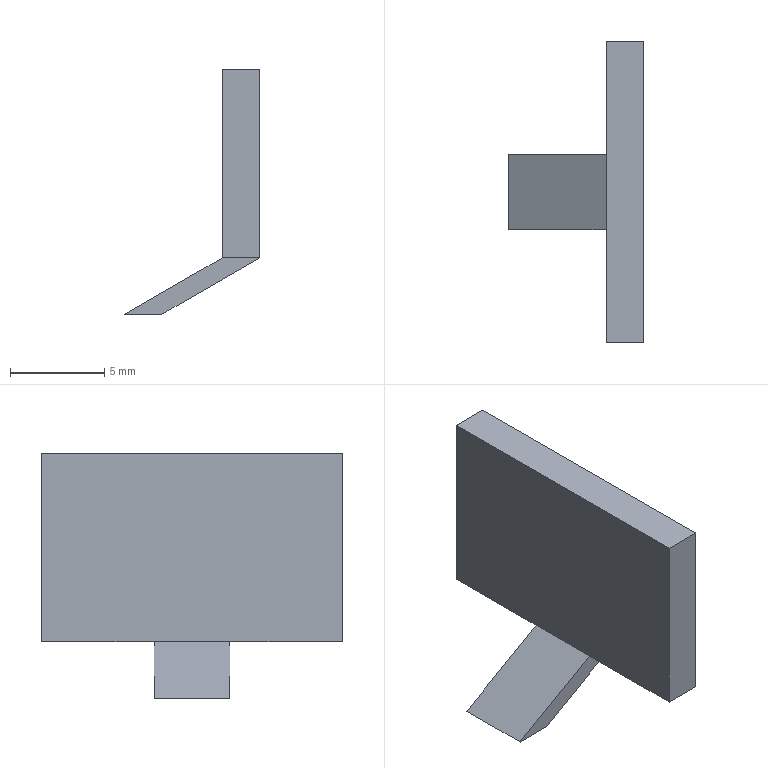Component | NX | GRIPPER_21 | 1 solid | 12 faces | box 7.2 x 16 x 12.99 mm | volume 344 mm3 | plane 12
STEP:
#1=CARTESIAN_POINT('',(0.,0.,0.));
#2=DIRECTION('',(0.,0.,1.));
#3=DIRECTION('',(1.,0.,0.));
#4=AXIS2_PLACEMENT_3D('',#1,#2,#3);
#5=CARTESIAN_POINT('',(26.071,12.637,119.668));
#6=VERTEX_POINT('',#5);
#7=CARTESIAN_POINT('',(24.071,12.637,119.668));
#8=VERTEX_POINT('',#7);
#9=CARTESIAN_POINT('',(26.071,12.637,119.668));
#10=DIRECTION('',(-1.,0.,0.));
#11=VECTOR('',#10,1.);
#12=LINE('',#9,#11);
#13=CARTESIAN_POINT('',(24.071,6.637,119.668));
#14=DIRECTION('',(0.,0.,1.));
#15=DIRECTION('',(-1.,0.,0.));
#16=AXIS2_PLACEMENT_3D('',#13,#14,#15);
#17=PLANE('',#16);
#18=CARTESIAN_POINT('',(-2.,-6.));
#19=DIRECTION('',(1.,0.));
#20=VECTOR('',#19,1.);
#21=LINE('',#18,#20);
#22=(GEOMETRIC_REPRESENTATION_CONTEXT(2)PARAMETRIC_REPRESENTATION_CONTEXT()REPRESENTATION_CONTEXT('',''));
#23=DEFINITIONAL_REPRESENTATION('',(#21),#22);
#24=PCURVE('',#17,#23);
#25=CARTESIAN_POINT('',(26.071,12.637,119.668));
#26=DIRECTION('',(0.,-1.,0.));
#27=DIRECTION('',(1.,0.,0.));
#28=AXIS2_PLACEMENT_3D('',#25,#26,#27);
#29=PLANE('',#28);
#30=CARTESIAN_POINT('',(0.,0.));
#31=DIRECTION('',(-1.,0.));
#32=VECTOR('',#31,1.);
#33=LINE('',#30,#32);
#34=(GEOMETRIC_REPRESENTATION_CONTEXT(2)PARAMETRIC_REPRESENTATION_CONTEXT()REPRESENTATION_CONTEXT('',''));
#35=DEFINITIONAL_REPRESENTATION('',(#33),#34);
#36=PCURVE('',#29,#35);
#37=SURFACE_CURVE('',#12,(#24,#36),.PCURVE_S1.);
#38=EDGE_CURVE('',#6,#8,#37,.T.);
#39=ORIENTED_EDGE('',*,*,#38,.F.);
#40=CARTESIAN_POINT('',(26.071,6.637,119.668));
#41=VERTEX_POINT('',#40);
#42=CARTESIAN_POINT('',(26.071,6.637,119.668));
#43=DIRECTION('',(0.,1.,0.));
#44=VECTOR('',#43,1.);
#45=LINE('',#42,#44);
#46=CARTESIAN_POINT('',(-2.,0.));
#47=DIRECTION('',(0.,-1.));
#48=VECTOR('',#47,1.);
#49=LINE('',#46,#48);
#50=(GEOMETRIC_REPRESENTATION_CONTEXT(2)PARAMETRIC_REPRESENTATION_CONTEXT()REPRESENTATION_CONTEXT('',''));
#51=DEFINITIONAL_REPRESENTATION('',(#49),#50);
#52=PCURVE('',#17,#51);
#53=CARTESIAN_POINT('',(26.071,6.637,119.668));
#54=DIRECTION('',(-1.,0.,0.));
#55=DIRECTION('',(0.,-1.,0.));
#56=AXIS2_PLACEMENT_3D('',#53,#54,#55);
#57=PLANE('',#56);
#58=CARTESIAN_POINT('',(0.,0.));
#59=DIRECTION('',(-1.,0.));
#60=VECTOR('',#59,1.);
#61=LINE('',#58,#60);
#62=(GEOMETRIC_REPRESENTATION_CONTEXT(2)PARAMETRIC_REPRESENTATION_CONTEXT()REPRESENTATION_CONTEXT('',''));
#63=DEFINITIONAL_REPRESENTATION('',(#61),#62);
#64=PCURVE('',#57,#63);
#65=SURFACE_CURVE('',#45,(#52,#64),.PCURVE_S1.);
#66=EDGE_CURVE('',#41,#6,#65,.T.);
#67=ORIENTED_EDGE('',*,*,#66,.F.);
#68=CARTESIAN_POINT('',(24.071,6.637,119.668));
#69=VERTEX_POINT('',#68);
#70=CARTESIAN_POINT('',(24.071,6.637,119.668));
#71=DIRECTION('',(1.,0.,-0.));
#72=VECTOR('',#71,1.);
#73=LINE('',#70,#72);
#74=CARTESIAN_POINT('',(0.,0.));
#75=DIRECTION('',(-1.,0.));
#76=VECTOR('',#75,1.);
#77=LINE('',#74,#76);
#78=(GEOMETRIC_REPRESENTATION_CONTEXT(2)PARAMETRIC_REPRESENTATION_CONTEXT()REPRESENTATION_CONTEXT('',''));
#79=DEFINITIONAL_REPRESENTATION('',(#77),#78);
#80=PCURVE('',#17,#79);
#81=CARTESIAN_POINT('',(26.071,6.637,119.668));
#82=DIRECTION('',(0.,-1.,0.));
#83=DIRECTION('',(1.,0.,0.));
#84=AXIS2_PLACEMENT_3D('',#81,#82,#83);
#85=PLANE('',#84);
#86=CARTESIAN_POINT('',(-2.,0.));
#87=DIRECTION('',(1.,-0.));
#88=VECTOR('',#87,1.);
#89=LINE('',#86,#88);
#90=(GEOMETRIC_REPRESENTATION_CONTEXT(2)PARAMETRIC_REPRESENTATION_CONTEXT()REPRESENTATION_CONTEXT('',''));
#91=DEFINITIONAL_REPRESENTATION('',(#89),#90);
#92=PCURVE('',#85,#91);
#93=SURFACE_CURVE('',#73,(#80,#92),.PCURVE_S1.);
#94=EDGE_CURVE('',#69,#41,#93,.T.);
#95=ORIENTED_EDGE('',*,*,#94,.F.);
#96=CARTESIAN_POINT('',(24.071,6.637,119.668));
#97=DIRECTION('',(0.,1.,0.));
#98=VECTOR('',#97,1.);
#99=LINE('',#96,#98);
#100=CARTESIAN_POINT('',(0.,0.));
#101=DIRECTION('',(0.,-1.));
#102=VECTOR('',#101,1.);
#103=LINE('',#100,#102);
#104=(GEOMETRIC_REPRESENTATION_CONTEXT(2)PARAMETRIC_REPRESENTATION_CONTEXT()REPRESENTATION_CONTEXT('',''));
#105=DEFINITIONAL_REPRESENTATION('',(#103),#104);
#106=PCURVE('',#17,#105);
#107=CARTESIAN_POINT('',(24.071,6.637,129.668));
#108=DIRECTION('',(1.,0.,0.));
#109=DIRECTION('',(-0.,0.,1.));
#110=AXIS2_PLACEMENT_3D('',#107,#108,#109);
#111=PLANE('',#110);
#112=CARTESIAN_POINT('',(-10.,0.));
#113=DIRECTION('',(0.,-1.));
#114=VECTOR('',#113,1.);
#115=LINE('',#112,#114);
#116=(GEOMETRIC_REPRESENTATION_CONTEXT(2)PARAMETRIC_REPRESENTATION_CONTEXT()REPRESENTATION_CONTEXT('',''));
#117=DEFINITIONAL_REPRESENTATION('',(#115),#116);
#118=PCURVE('',#111,#117);
#119=SURFACE_CURVE('',#99,(#106,#118),.PCURVE_S1.);
#120=EDGE_CURVE('',#69,#8,#119,.T.);
#121=ORIENTED_EDGE('',*,*,#120,.T.);
#122=EDGE_LOOP('',(#39,#67,#95,#121));
#123=FACE_BOUND('',#122,.T.);
#124=ADVANCED_FACE('',(#123),#17,.F.);
#125=CARTESIAN_POINT('',(26.071,22.637,119.668));
#126=VERTEX_POINT('',#125);
#127=CARTESIAN_POINT('',(26.071,22.637,129.668));
#128=VERTEX_POINT('',#127);
#129=CARTESIAN_POINT('',(26.071,22.637,119.668));
#130=DIRECTION('',(0.,0.,1.));
#131=VECTOR('',#130,1.);
#132=LINE('',#129,#131);
#133=CARTESIAN_POINT('',(-16.,0.));
#134=DIRECTION('',(0.,1.));
#135=VECTOR('',#134,1.);
#136=LINE('',#133,#135);
#137=(GEOMETRIC_REPRESENTATION_CONTEXT(2)PARAMETRIC_REPRESENTATION_CONTEXT()REPRESENTATION_CONTEXT('',''));
#138=DEFINITIONAL_REPRESENTATION('',(#136),#137);
#139=PCURVE('',#57,#138);
#140=CARTESIAN_POINT('',(26.071,22.637,119.668));
#141=DIRECTION('',(0.,-1.,0.));
#142=DIRECTION('',(1.,0.,0.));
#143=AXIS2_PLACEMENT_3D('',#140,#141,#142);
#144=PLANE('',#143);
#145=CARTESIAN_POINT('',(0.,0.));
#146=DIRECTION('',(0.,1.));
#147=VECTOR('',#146,1.);
#148=LINE('',#145,#147);
#149=(GEOMETRIC_REPRESENTATION_CONTEXT(2)PARAMETRIC_REPRESENTATION_CONTEXT()REPRESENTATION_CONTEXT('',''));
#150=DEFINITIONAL_REPRESENTATION('',(#148),#149);
#151=PCURVE('',#144,#150);
#152=SURFACE_CURVE('',#132,(#139,#151),.PCURVE_S1.);
#153=EDGE_CURVE('',#126,#128,#152,.T.);
#154=ORIENTED_EDGE('',*,*,#153,.T.);
#155=CARTESIAN_POINT('',(26.071,6.637,129.668));
#156=VERTEX_POINT('',#155);
#157=CARTESIAN_POINT('',(26.071,6.637,129.668));
#158=DIRECTION('',(0.,1.,0.));
#159=VECTOR('',#158,1.);
#160=LINE('',#157,#159);
#161=CARTESIAN_POINT('',(0.,10.));
#162=DIRECTION('',(-1.,0.));
#163=VECTOR('',#162,1.);
#164=LINE('',#161,#163);
#165=(GEOMETRIC_REPRESENTATION_CONTEXT(2)PARAMETRIC_REPRESENTATION_CONTEXT()REPRESENTATION_CONTEXT('',''));
#166=DEFINITIONAL_REPRESENTATION('',(#164),#165);
#167=PCURVE('',#57,#166);
#168=CARTESIAN_POINT('',(26.071,6.637,129.668));
#169=DIRECTION('',(-0.,0.,-1.));
#170=DIRECTION('',(1.,0.,-0.));
#171=AXIS2_PLACEMENT_3D('',#168,#169,#170);
#172=PLANE('',#171);
#173=CARTESIAN_POINT('',(0.,0.));
#174=DIRECTION('',(0.,-1.));
#175=VECTOR('',#174,1.);
#176=LINE('',#173,#175);
#177=(GEOMETRIC_REPRESENTATION_CONTEXT(2)PARAMETRIC_REPRESENTATION_CONTEXT()REPRESENTATION_CONTEXT('',''));
#178=DEFINITIONAL_REPRESENTATION('',(#176),#177);
#179=PCURVE('',#172,#178);
#180=SURFACE_CURVE('',#160,(#167,#179),.PCURVE_S1.);
#181=EDGE_CURVE('',#156,#128,#180,.T.);
#182=ORIENTED_EDGE('',*,*,#181,.F.);
#183=CARTESIAN_POINT('',(26.071,6.637,119.668));
#184=DIRECTION('',(0.,0.,1.));
#185=VECTOR('',#184,1.);
#186=LINE('',#183,#185);
#187=CARTESIAN_POINT('',(0.,0.));
#188=DIRECTION('',(0.,1.));
#189=VECTOR('',#188,1.);
#190=LINE('',#187,#189);
#191=(GEOMETRIC_REPRESENTATION_CONTEXT(2)PARAMETRIC_REPRESENTATION_CONTEXT()REPRESENTATION_CONTEXT('',''));
#192=DEFINITIONAL_REPRESENTATION('',(#190),#191);
#193=PCURVE('',#57,#192);
#194=CARTESIAN_POINT('',(0.,0.));
#195=DIRECTION('',(0.,1.));
#196=VECTOR('',#195,1.);
#197=LINE('',#194,#196);
#198=(GEOMETRIC_REPRESENTATION_CONTEXT(2)PARAMETRIC_REPRESENTATION_CONTEXT()REPRESENTATION_CONTEXT('',''));
#199=DEFINITIONAL_REPRESENTATION('',(#197),#198);
#200=PCURVE('',#85,#199);
#201=SURFACE_CURVE('',#186,(#193,#200),.PCURVE_S1.);
#202=EDGE_CURVE('',#41,#156,#201,.T.);
#203=ORIENTED_EDGE('',*,*,#202,.F.);
#204=ORIENTED_EDGE('',*,*,#66,.T.);
#205=CARTESIAN_POINT('',(26.071,16.637,119.668));
#206=VERTEX_POINT('',#205);
#207=CARTESIAN_POINT('',(26.071,12.637,119.668));
#208=DIRECTION('',(0.,1.,0.));
#209=VECTOR('',#208,1.);
#210=LINE('',#207,#209);
#211=CARTESIAN_POINT('',(-6.,0.));
#212=DIRECTION('',(-1.,0.));
#213=VECTOR('',#212,1.);
#214=LINE('',#211,#213);
#215=(GEOMETRIC_REPRESENTATION_CONTEXT(2)PARAMETRIC_REPRESENTATION_CONTEXT()REPRESENTATION_CONTEXT('',''));
#216=DEFINITIONAL_REPRESENTATION('',(#214),#215);
#217=PCURVE('',#57,#216);
#218=CARTESIAN_POINT('',(20.871,12.637,116.674));
#219=DIRECTION('',(-0.4989,0.,0.8667));
#220=DIRECTION('',(-0.8667,0.,-0.4989));
#221=AXIS2_PLACEMENT_3D('',#218,#219,#220);
#222=PLANE('',#221);
#223=CARTESIAN_POINT('',(-6.,0.));
#224=DIRECTION('',(0.,-1.));
#225=VECTOR('',#224,1.);
#226=LINE('',#223,#225);
#227=(GEOMETRIC_REPRESENTATION_CONTEXT(2)PARAMETRIC_REPRESENTATION_CONTEXT()REPRESENTATION_CONTEXT('',''));
#228=DEFINITIONAL_REPRESENTATION('',(#226),#227);
#229=PCURVE('',#222,#228);
#230=SURFACE_CURVE('',#210,(#217,#229),.PCURVE_S1.);
#231=EDGE_CURVE('',#6,#206,#230,.T.);
#232=ORIENTED_EDGE('',*,*,#231,.T.);
#233=CARTESIAN_POINT('',(26.071,6.637,119.668));
#234=DIRECTION('',(0.,1.,0.));
#235=VECTOR('',#234,1.);
#236=LINE('',#233,#235);
#237=CARTESIAN_POINT('',(0.,0.));
#238=DIRECTION('',(-1.,0.));
#239=VECTOR('',#238,1.);
#240=LINE('',#237,#239);
#241=(GEOMETRIC_REPRESENTATION_CONTEXT(2)PARAMETRIC_REPRESENTATION_CONTEXT()REPRESENTATION_CONTEXT('',''));
#242=DEFINITIONAL_REPRESENTATION('',(#240),#241);
#243=PCURVE('',#57,#242);
#244=CARTESIAN_POINT('',(24.071,6.637,119.668));
#245=DIRECTION('',(0.,0.,1.));
#246=DIRECTION('',(-1.,0.,0.));
#247=AXIS2_PLACEMENT_3D('',#244,#245,#246);
#248=PLANE('',#247);
#249=CARTESIAN_POINT('',(-2.,0.));
#250=DIRECTION('',(0.,-1.));
#251=VECTOR('',#250,1.);
#252=LINE('',#249,#251);
#253=(GEOMETRIC_REPRESENTATION_CONTEXT(2)PARAMETRIC_REPRESENTATION_CONTEXT()REPRESENTATION_CONTEXT('',''));
#254=DEFINITIONAL_REPRESENTATION('',(#252),#253);
#255=PCURVE('',#248,#254);
#256=SURFACE_CURVE('',#236,(#243,#255),.PCURVE_S1.);
#257=EDGE_CURVE('',#206,#126,#256,.T.);
#258=ORIENTED_EDGE('',*,*,#257,.T.);
#259=EDGE_LOOP('',(#154,#182,#203,#204,#232,#258));
#260=FACE_BOUND('',#259,.T.);
#261=ADVANCED_FACE('',(#260),#57,.F.);
#262=CARTESIAN_POINT('',(24.071,22.637,129.668));
#263=VERTEX_POINT('',#262);
#264=CARTESIAN_POINT('',(26.071,22.637,129.668));
#265=DIRECTION('',(-1.,0.,0.));
#266=VECTOR('',#265,1.);
#267=LINE('',#264,#266);
#268=CARTESIAN_POINT('',(0.,-16.));
#269=DIRECTION('',(-1.,0.));
#270=VECTOR('',#269,1.);
#271=LINE('',#268,#270);
#272=(GEOMETRIC_REPRESENTATION_CONTEXT(2)PARAMETRIC_REPRESENTATION_CONTEXT()REPRESENTATION_CONTEXT('',''));
#273=DEFINITIONAL_REPRESENTATION('',(#271),#272);
#274=PCURVE('',#172,#273);
#275=CARTESIAN_POINT('',(0.,10.));
#276=DIRECTION('',(-1.,0.));
#277=VECTOR('',#276,1.);
#278=LINE('',#275,#277);
#279=(GEOMETRIC_REPRESENTATION_CONTEXT(2)PARAMETRIC_REPRESENTATION_CONTEXT()REPRESENTATION_CONTEXT('',''));
#280=DEFINITIONAL_REPRESENTATION('',(#278),#279);
#281=PCURVE('',#144,#280);
#282=SURFACE_CURVE('',#267,(#274,#281),.PCURVE_S1.);
#283=EDGE_CURVE('',#128,#263,#282,.T.);
#284=ORIENTED_EDGE('',*,*,#283,.T.);
#285=CARTESIAN_POINT('',(24.071,6.637,129.668));
#286=VERTEX_POINT('',#285);
#287=CARTESIAN_POINT('',(24.071,6.637,129.668));
#288=DIRECTION('',(0.,1.,0.));
#289=VECTOR('',#288,1.);
#290=LINE('',#287,#289);
#291=CARTESIAN_POINT('',(-2.,0.));
#292=DIRECTION('',(0.,-1.));
#293=VECTOR('',#292,1.);
#294=LINE('',#291,#293);
#295=(GEOMETRIC_REPRESENTATION_CONTEXT(2)PARAMETRIC_REPRESENTATION_CONTEXT()REPRESENTATION_CONTEXT('',''));
#296=DEFINITIONAL_REPRESENTATION('',(#294),#295);
#297=PCURVE('',#172,#296);
#298=CARTESIAN_POINT('',(0.,0.));
#299=DIRECTION('',(0.,-1.));
#300=VECTOR('',#299,1.);
#301=LINE('',#298,#300);
#302=(GEOMETRIC_REPRESENTATION_CONTEXT(2)PARAMETRIC_REPRESENTATION_CONTEXT()REPRESENTATION_CONTEXT('',''));
#303=DEFINITIONAL_REPRESENTATION('',(#301),#302);
#304=PCURVE('',#111,#303);
#305=SURFACE_CURVE('',#290,(#297,#304),.PCURVE_S1.);
#306=EDGE_CURVE('',#286,#263,#305,.T.);
#307=ORIENTED_EDGE('',*,*,#306,.F.);
#308=CARTESIAN_POINT('',(26.071,6.637,129.668));
#309=DIRECTION('',(-1.,0.,0.));
#310=VECTOR('',#309,1.);
#311=LINE('',#308,#310);
#312=CARTESIAN_POINT('',(0.,0.));
#313=DIRECTION('',(-1.,0.));
#314=VECTOR('',#313,1.);
#315=LINE('',#312,#314);
#316=(GEOMETRIC_REPRESENTATION_CONTEXT(2)PARAMETRIC_REPRESENTATION_CONTEXT()REPRESENTATION_CONTEXT('',''));
#317=DEFINITIONAL_REPRESENTATION('',(#315),#316);
#318=PCURVE('',#172,#317);
#319=CARTESIAN_POINT('',(0.,10.));
#320=DIRECTION('',(-1.,0.));
#321=VECTOR('',#320,1.);
#322=LINE('',#319,#321);
#323=(GEOMETRIC_REPRESENTATION_CONTEXT(2)PARAMETRIC_REPRESENTATION_CONTEXT()REPRESENTATION_CONTEXT('',''));
#324=DEFINITIONAL_REPRESENTATION('',(#322),#323);
#325=PCURVE('',#85,#324);
#326=SURFACE_CURVE('',#311,(#318,#325),.PCURVE_S1.);
#327=EDGE_CURVE('',#156,#286,#326,.T.);
#328=ORIENTED_EDGE('',*,*,#327,.F.);
#329=ORIENTED_EDGE('',*,*,#181,.T.);
#330=EDGE_LOOP('',(#284,#307,#328,#329));
#331=FACE_BOUND('',#330,.T.);
#332=ADVANCED_FACE('',(#331),#172,.F.);
#333=CARTESIAN_POINT('',(24.071,22.637,119.668));
#334=VERTEX_POINT('',#333);
#335=CARTESIAN_POINT('',(24.071,22.637,129.668));
#336=DIRECTION('',(0.,0.,-1.));
#337=VECTOR('',#336,1.);
#338=LINE('',#335,#337);
#339=CARTESIAN_POINT('',(0.,-16.));
#340=DIRECTION('',(-1.,0.));
#341=VECTOR('',#340,1.);
#342=LINE('',#339,#341);
#343=(GEOMETRIC_REPRESENTATION_CONTEXT(2)PARAMETRIC_REPRESENTATION_CONTEXT()REPRESENTATION_CONTEXT('',''));
#344=DEFINITIONAL_REPRESENTATION('',(#342),#343);
#345=PCURVE('',#111,#344);
#346=CARTESIAN_POINT('',(-2.,10.));
#347=DIRECTION('',(0.,-1.));
#348=VECTOR('',#347,1.);
#349=LINE('',#346,#348);
#350=(GEOMETRIC_REPRESENTATION_CONTEXT(2)PARAMETRIC_REPRESENTATION_CONTEXT()REPRESENTATION_CONTEXT('',''));
#351=DEFINITIONAL_REPRESENTATION('',(#349),#350);
#352=PCURVE('',#144,#351);
#353=SURFACE_CURVE('',#338,(#345,#352),.PCURVE_S1.);
#354=EDGE_CURVE('',#263,#334,#353,.T.);
#355=ORIENTED_EDGE('',*,*,#354,.T.);
#356=CARTESIAN_POINT('',(24.071,16.637,119.668));
#357=VERTEX_POINT('',#356);
#358=CARTESIAN_POINT('',(24.071,6.637,119.668));
#359=DIRECTION('',(0.,1.,0.));
#360=VECTOR('',#359,1.);
#361=LINE('',#358,#360);
#362=CARTESIAN_POINT('',(-10.,0.));
#363=DIRECTION('',(0.,-1.));
#364=VECTOR('',#363,1.);
#365=LINE('',#362,#364);
#366=(GEOMETRIC_REPRESENTATION_CONTEXT(2)PARAMETRIC_REPRESENTATION_CONTEXT()REPRESENTATION_CONTEXT('',''));
#367=DEFINITIONAL_REPRESENTATION('',(#365),#366);
#368=PCURVE('',#111,#367);
#369=CARTESIAN_POINT('',(0.,0.));
#370=DIRECTION('',(0.,-1.));
#371=VECTOR('',#370,1.);
#372=LINE('',#369,#371);
#373=(GEOMETRIC_REPRESENTATION_CONTEXT(2)PARAMETRIC_REPRESENTATION_CONTEXT()REPRESENTATION_CONTEXT('',''));
#374=DEFINITIONAL_REPRESENTATION('',(#372),#373);
#375=PCURVE('',#248,#374);
#376=SURFACE_CURVE('',#361,(#368,#375),.PCURVE_S1.);
#377=EDGE_CURVE('',#357,#334,#376,.T.);
#378=ORIENTED_EDGE('',*,*,#377,.F.);
#379=CARTESIAN_POINT('',(24.071,12.637,119.668));
#380=DIRECTION('',(0.,1.,0.));
#381=VECTOR('',#380,1.);
#382=LINE('',#379,#381);
#383=CARTESIAN_POINT('',(-10.,-6.));
#384=DIRECTION('',(0.,-1.));
#385=VECTOR('',#384,1.);
#386=LINE('',#383,#385);
#387=(GEOMETRIC_REPRESENTATION_CONTEXT(2)PARAMETRIC_REPRESENTATION_CONTEXT()REPRESENTATION_CONTEXT('',''));
#388=DEFINITIONAL_REPRESENTATION('',(#386),#387);
#389=PCURVE('',#111,#388);
#390=CARTESIAN_POINT('',(24.071,12.637,119.668));
#391=DIRECTION('',(0.4989,0.,-0.8667));
#392=DIRECTION('',(0.8667,0.,0.4989));
#393=AXIS2_PLACEMENT_3D('',#390,#391,#392);
#394=PLANE('',#393);
#395=CARTESIAN_POINT('',(0.,0.));
#396=DIRECTION('',(0.,-1.));
#397=VECTOR('',#396,1.);
#398=LINE('',#395,#397);
#399=(GEOMETRIC_REPRESENTATION_CONTEXT(2)PARAMETRIC_REPRESENTATION_CONTEXT()REPRESENTATION_CONTEXT('',''));
#400=DEFINITIONAL_REPRESENTATION('',(#398),#399);
#401=PCURVE('',#394,#400);
#402=SURFACE_CURVE('',#382,(#389,#401),.PCURVE_S1.);
#403=EDGE_CURVE('',#8,#357,#402,.T.);
#404=ORIENTED_EDGE('',*,*,#403,.F.);
#405=ORIENTED_EDGE('',*,*,#120,.F.);
#406=CARTESIAN_POINT('',(24.071,6.637,129.668));
#407=DIRECTION('',(0.,0.,-1.));
#408=VECTOR('',#407,1.);
#409=LINE('',#406,#408);
#410=CARTESIAN_POINT('',(0.,0.));
#411=DIRECTION('',(-1.,0.));
#412=VECTOR('',#411,1.);
#413=LINE('',#410,#412);
#414=(GEOMETRIC_REPRESENTATION_CONTEXT(2)PARAMETRIC_REPRESENTATION_CONTEXT()REPRESENTATION_CONTEXT('',''));
#415=DEFINITIONAL_REPRESENTATION('',(#413),#414);
#416=PCURVE('',#111,#415);
#417=CARTESIAN_POINT('',(-2.,10.));
#418=DIRECTION('',(0.,-1.));
#419=VECTOR('',#418,1.);
#420=LINE('',#417,#419);
#421=(GEOMETRIC_REPRESENTATION_CONTEXT(2)PARAMETRIC_REPRESENTATION_CONTEXT()REPRESENTATION_CONTEXT('',''));
#422=DEFINITIONAL_REPRESENTATION('',(#420),#421);
#423=PCURVE('',#85,#422);
#424=SURFACE_CURVE('',#409,(#416,#423),.PCURVE_S1.);
#425=EDGE_CURVE('',#286,#69,#424,.T.);
#426=ORIENTED_EDGE('',*,*,#425,.F.);
#427=ORIENTED_EDGE('',*,*,#306,.T.);
#428=EDGE_LOOP('',(#355,#378,#404,#405,#426,#427));
#429=FACE_BOUND('',#428,.T.);
#430=ADVANCED_FACE('',(#429),#111,.F.);
#431=ORIENTED_EDGE('',*,*,#257,.F.);
#432=CARTESIAN_POINT('',(26.071,16.637,119.668));
#433=DIRECTION('',(-1.,0.,0.));
#434=VECTOR('',#433,1.);
#435=LINE('',#432,#434);
#436=CARTESIAN_POINT('',(-2.,-10.));
#437=DIRECTION('',(1.,0.));
#438=VECTOR('',#437,1.);
#439=LINE('',#436,#438);
#440=(GEOMETRIC_REPRESENTATION_CONTEXT(2)PARAMETRIC_REPRESENTATION_CONTEXT()REPRESENTATION_CONTEXT('',''));
#441=DEFINITIONAL_REPRESENTATION('',(#439),#440);
#442=PCURVE('',#248,#441);
#443=CARTESIAN_POINT('',(26.071,16.637,119.668));
#444=DIRECTION('',(0.,-1.,0.));
#445=DIRECTION('',(1.,0.,0.));
#446=AXIS2_PLACEMENT_3D('',#443,#444,#445);
#447=PLANE('',#446);
#448=CARTESIAN_POINT('',(0.,0.));
#449=DIRECTION('',(-1.,0.));
#450=VECTOR('',#449,1.);
#451=LINE('',#448,#450);
#452=(GEOMETRIC_REPRESENTATION_CONTEXT(2)PARAMETRIC_REPRESENTATION_CONTEXT()REPRESENTATION_CONTEXT('',''));
#453=DEFINITIONAL_REPRESENTATION('',(#451),#452);
#454=PCURVE('',#447,#453);
#455=SURFACE_CURVE('',#435,(#442,#454),.PCURVE_S1.);
#456=EDGE_CURVE('',#206,#357,#455,.T.);
#457=ORIENTED_EDGE('',*,*,#456,.T.);
#458=ORIENTED_EDGE('',*,*,#377,.T.);
#459=CARTESIAN_POINT('',(24.071,22.637,119.668));
#460=DIRECTION('',(1.,0.,-0.));
#461=VECTOR('',#460,1.);
#462=LINE('',#459,#461);
#463=CARTESIAN_POINT('',(0.,-16.));
#464=DIRECTION('',(-1.,0.));
#465=VECTOR('',#464,1.);
#466=LINE('',#463,#465);
#467=(GEOMETRIC_REPRESENTATION_CONTEXT(2)PARAMETRIC_REPRESENTATION_CONTEXT()REPRESENTATION_CONTEXT('',''));
#468=DEFINITIONAL_REPRESENTATION('',(#466),#467);
#469=PCURVE('',#248,#468);
#470=CARTESIAN_POINT('',(-2.,0.));
#471=DIRECTION('',(1.,-0.));
#472=VECTOR('',#471,1.);
#473=LINE('',#470,#472);
#474=(GEOMETRIC_REPRESENTATION_CONTEXT(2)PARAMETRIC_REPRESENTATION_CONTEXT()REPRESENTATION_CONTEXT('',''));
#475=DEFINITIONAL_REPRESENTATION('',(#473),#474);
#476=PCURVE('',#144,#475);
#477=SURFACE_CURVE('',#462,(#469,#476),.PCURVE_S1.);
#478=EDGE_CURVE('',#334,#126,#477,.T.);
#479=ORIENTED_EDGE('',*,*,#478,.T.);
#480=EDGE_LOOP('',(#431,#457,#458,#479));
#481=FACE_BOUND('',#480,.T.);
#482=ADVANCED_FACE('',(#481),#248,.F.);
#483=ORIENTED_EDGE('',*,*,#202,.T.);
#484=ORIENTED_EDGE('',*,*,#327,.T.);
#485=ORIENTED_EDGE('',*,*,#425,.T.);
#486=ORIENTED_EDGE('',*,*,#94,.T.);
#487=EDGE_LOOP('',(#483,#484,#485,#486));
#488=FACE_BOUND('',#487,.T.);
#489=ADVANCED_FACE('',(#488),#85,.T.);
#490=ORIENTED_EDGE('',*,*,#153,.F.);
#491=ORIENTED_EDGE('',*,*,#478,.F.);
#492=ORIENTED_EDGE('',*,*,#354,.F.);
#493=ORIENTED_EDGE('',*,*,#283,.F.);
#494=EDGE_LOOP('',(#490,#491,#492,#493));
#495=FACE_BOUND('',#494,.T.);
#496=ADVANCED_FACE('',(#495),#144,.F.);
#497=CARTESIAN_POINT('',(18.871,16.637,116.674));
#498=VERTEX_POINT('',#497);
#499=CARTESIAN_POINT('',(20.871,16.637,116.674));
#500=VERTEX_POINT('',#499);
#501=CARTESIAN_POINT('',(18.871,16.637,116.674));
#502=DIRECTION('',(1.,0.,0.));
#503=VECTOR('',#502,1.);
#504=LINE('',#501,#503);
#505=CARTESIAN_POINT('',(18.871,12.637,116.674));
#506=DIRECTION('',(0.,0.,1.));
#507=DIRECTION('',(-1.,0.,0.));
#508=AXIS2_PLACEMENT_3D('',#505,#506,#507);
#509=PLANE('',#508);
#510=CARTESIAN_POINT('',(0.,-4.));
#511=DIRECTION('',(-1.,0.));
#512=VECTOR('',#511,1.);
#513=LINE('',#510,#512);
#514=(GEOMETRIC_REPRESENTATION_CONTEXT(2)PARAMETRIC_REPRESENTATION_CONTEXT()REPRESENTATION_CONTEXT('',''));
#515=DEFINITIONAL_REPRESENTATION('',(#513),#514);
#516=PCURVE('',#509,#515);
#517=CARTESIAN_POINT('',(-7.2,-2.993));
#518=DIRECTION('',(1.,0.));
#519=VECTOR('',#518,1.);
#520=LINE('',#517,#519);
#521=(GEOMETRIC_REPRESENTATION_CONTEXT(2)PARAMETRIC_REPRESENTATION_CONTEXT()REPRESENTATION_CONTEXT('',''));
#522=DEFINITIONAL_REPRESENTATION('',(#520),#521);
#523=PCURVE('',#447,#522);
#524=SURFACE_CURVE('',#504,(#516,#523),.PCURVE_S1.);
#525=EDGE_CURVE('',#498,#500,#524,.T.);
#526=ORIENTED_EDGE('',*,*,#525,.T.);
#527=CARTESIAN_POINT('',(20.871,12.637,116.674));
#528=VERTEX_POINT('',#527);
#529=CARTESIAN_POINT('',(20.871,12.637,116.674));
#530=DIRECTION('',(0.,1.,0.));
#531=VECTOR('',#530,1.);
#532=LINE('',#529,#531);
#533=CARTESIAN_POINT('',(-2.,0.));
#534=DIRECTION('',(0.,-1.));
#535=VECTOR('',#534,1.);
#536=LINE('',#533,#535);
#537=(GEOMETRIC_REPRESENTATION_CONTEXT(2)PARAMETRIC_REPRESENTATION_CONTEXT()REPRESENTATION_CONTEXT('',''));
#538=DEFINITIONAL_REPRESENTATION('',(#536),#537);
#539=PCURVE('',#509,#538);
#540=CARTESIAN_POINT('',(0.,0.));
#541=DIRECTION('',(0.,-1.));
#542=VECTOR('',#541,1.);
#543=LINE('',#540,#542);
#544=(GEOMETRIC_REPRESENTATION_CONTEXT(2)PARAMETRIC_REPRESENTATION_CONTEXT()REPRESENTATION_CONTEXT('',''));
#545=DEFINITIONAL_REPRESENTATION('',(#543),#544);
#546=PCURVE('',#222,#545);
#547=SURFACE_CURVE('',#532,(#539,#546),.PCURVE_S1.);
#548=EDGE_CURVE('',#528,#500,#547,.T.);
#549=ORIENTED_EDGE('',*,*,#548,.F.);
#550=CARTESIAN_POINT('',(18.871,12.637,116.674));
#551=VERTEX_POINT('',#550);
#552=CARTESIAN_POINT('',(18.871,12.637,116.674));
#553=DIRECTION('',(1.,0.,0.));
#554=VECTOR('',#553,1.);
#555=LINE('',#552,#554);
#556=CARTESIAN_POINT('',(0.,0.));
#557=DIRECTION('',(-1.,0.));
#558=VECTOR('',#557,1.);
#559=LINE('',#556,#558);
#560=(GEOMETRIC_REPRESENTATION_CONTEXT(2)PARAMETRIC_REPRESENTATION_CONTEXT()REPRESENTATION_CONTEXT('',''));
#561=DEFINITIONAL_REPRESENTATION('',(#559),#560);
#562=PCURVE('',#509,#561);
#563=CARTESIAN_POINT('',(-7.2,-2.993));
#564=DIRECTION('',(1.,0.));
#565=VECTOR('',#564,1.);
#566=LINE('',#563,#565);
#567=(GEOMETRIC_REPRESENTATION_CONTEXT(2)PARAMETRIC_REPRESENTATION_CONTEXT()REPRESENTATION_CONTEXT('',''));
#568=DEFINITIONAL_REPRESENTATION('',(#566),#567);
#569=PCURVE('',#29,#568);
#570=SURFACE_CURVE('',#555,(#562,#569),.PCURVE_S1.);
#571=EDGE_CURVE('',#551,#528,#570,.T.);
#572=ORIENTED_EDGE('',*,*,#571,.F.);
#573=CARTESIAN_POINT('',(18.871,12.637,116.674));
#574=DIRECTION('',(0.,1.,0.));
#575=VECTOR('',#574,1.);
#576=LINE('',#573,#575);
#577=CARTESIAN_POINT('',(0.,0.));
#578=DIRECTION('',(0.,-1.));
#579=VECTOR('',#578,1.);
#580=LINE('',#577,#579);
#581=(GEOMETRIC_REPRESENTATION_CONTEXT(2)PARAMETRIC_REPRESENTATION_CONTEXT()REPRESENTATION_CONTEXT('',''));
#582=DEFINITIONAL_REPRESENTATION('',(#580),#581);
#583=PCURVE('',#509,#582);
#584=CARTESIAN_POINT('',(-6.,0.));
#585=DIRECTION('',(0.,-1.));
#586=VECTOR('',#585,1.);
#587=LINE('',#584,#586);
#588=(GEOMETRIC_REPRESENTATION_CONTEXT(2)PARAMETRIC_REPRESENTATION_CONTEXT()REPRESENTATION_CONTEXT('',''));
#589=DEFINITIONAL_REPRESENTATION('',(#587),#588);
#590=PCURVE('',#394,#589);
#591=SURFACE_CURVE('',#576,(#583,#590),.PCURVE_S1.);
#592=EDGE_CURVE('',#551,#498,#591,.T.);
#593=ORIENTED_EDGE('',*,*,#592,.T.);
#594=EDGE_LOOP('',(#526,#549,#572,#593));
#595=FACE_BOUND('',#594,.T.);
#596=ADVANCED_FACE('',(#595),#509,.F.);
#597=CARTESIAN_POINT('',(20.871,16.637,116.674));
#598=DIRECTION('',(0.8667,0.,0.4989));
#599=VECTOR('',#598,1.);
#600=LINE('',#597,#599);
#601=CARTESIAN_POINT('',(0.,-4.));
#602=DIRECTION('',(-1.,0.));
#603=VECTOR('',#602,1.);
#604=LINE('',#601,#603);
#605=(GEOMETRIC_REPRESENTATION_CONTEXT(2)PARAMETRIC_REPRESENTATION_CONTEXT()REPRESENTATION_CONTEXT('',''));
#606=DEFINITIONAL_REPRESENTATION('',(#604),#605);
#607=PCURVE('',#222,#606);
#608=CARTESIAN_POINT('',(-5.2,-2.993));
#609=DIRECTION('',(0.8667,0.4989));
#610=VECTOR('',#609,1.);
#611=LINE('',#608,#610);
#612=(GEOMETRIC_REPRESENTATION_CONTEXT(2)PARAMETRIC_REPRESENTATION_CONTEXT()REPRESENTATION_CONTEXT('',''));
#613=DEFINITIONAL_REPRESENTATION('',(#611),#612);
#614=PCURVE('',#447,#613);
#615=SURFACE_CURVE('',#600,(#607,#614),.PCURVE_S1.);
#616=EDGE_CURVE('',#500,#206,#615,.T.);
#617=ORIENTED_EDGE('',*,*,#616,.T.);
#618=ORIENTED_EDGE('',*,*,#231,.F.);
#619=CARTESIAN_POINT('',(20.871,12.637,116.674));
#620=DIRECTION('',(0.8667,0.,0.4989));
#621=VECTOR('',#620,1.);
#622=LINE('',#619,#621);
#623=CARTESIAN_POINT('',(0.,0.));
#624=DIRECTION('',(-1.,0.));
#625=VECTOR('',#624,1.);
#626=LINE('',#623,#625);
#627=(GEOMETRIC_REPRESENTATION_CONTEXT(2)PARAMETRIC_REPRESENTATION_CONTEXT()REPRESENTATION_CONTEXT('',''));
#628=DEFINITIONAL_REPRESENTATION('',(#626),#627);
#629=PCURVE('',#222,#628);
#630=CARTESIAN_POINT('',(-5.2,-2.993));
#631=DIRECTION('',(0.8667,0.4989));
#632=VECTOR('',#631,1.);
#633=LINE('',#630,#632);
#634=(GEOMETRIC_REPRESENTATION_CONTEXT(2)PARAMETRIC_REPRESENTATION_CONTEXT()REPRESENTATION_CONTEXT('',''));
#635=DEFINITIONAL_REPRESENTATION('',(#633),#634);
#636=PCURVE('',#29,#635);
#637=SURFACE_CURVE('',#622,(#629,#636),.PCURVE_S1.);
#638=EDGE_CURVE('',#528,#6,#637,.T.);
#639=ORIENTED_EDGE('',*,*,#638,.F.);
#640=ORIENTED_EDGE('',*,*,#548,.T.);
#641=EDGE_LOOP('',(#617,#618,#639,#640));
#642=FACE_BOUND('',#641,.T.);
#643=ADVANCED_FACE('',(#642),#222,.F.);
#644=CARTESIAN_POINT('',(24.071,16.637,119.668));
#645=DIRECTION('',(-0.8667,0.,-0.4989));
#646=VECTOR('',#645,1.);
#647=LINE('',#644,#646);
#648=CARTESIAN_POINT('',(0.,-4.));
#649=DIRECTION('',(-1.,0.));
#650=VECTOR('',#649,1.);
#651=LINE('',#648,#650);
#652=(GEOMETRIC_REPRESENTATION_CONTEXT(2)PARAMETRIC_REPRESENTATION_CONTEXT()REPRESENTATION_CONTEXT('',''));
#653=DEFINITIONAL_REPRESENTATION('',(#651),#652);
#654=PCURVE('',#394,#653);
#655=CARTESIAN_POINT('',(-2.,0.));
#656=DIRECTION('',(-0.8667,-0.4989));
#657=VECTOR('',#656,1.);
#658=LINE('',#655,#657);
#659=(GEOMETRIC_REPRESENTATION_CONTEXT(2)PARAMETRIC_REPRESENTATION_CONTEXT()REPRESENTATION_CONTEXT('',''));
#660=DEFINITIONAL_REPRESENTATION('',(#658),#659);
#661=PCURVE('',#447,#660);
#662=SURFACE_CURVE('',#647,(#654,#661),.PCURVE_S1.);
#663=EDGE_CURVE('',#357,#498,#662,.T.);
#664=ORIENTED_EDGE('',*,*,#663,.T.);
#665=ORIENTED_EDGE('',*,*,#592,.F.);
#666=CARTESIAN_POINT('',(24.071,12.637,119.668));
#667=DIRECTION('',(-0.8667,0.,-0.4989));
#668=VECTOR('',#667,1.);
#669=LINE('',#666,#668);
#670=CARTESIAN_POINT('',(0.,0.));
#671=DIRECTION('',(-1.,0.));
#672=VECTOR('',#671,1.);
#673=LINE('',#670,#672);
#674=(GEOMETRIC_REPRESENTATION_CONTEXT(2)PARAMETRIC_REPRESENTATION_CONTEXT()REPRESENTATION_CONTEXT('',''));
#675=DEFINITIONAL_REPRESENTATION('',(#673),#674);
#676=PCURVE('',#394,#675);
#677=CARTESIAN_POINT('',(-2.,0.));
#678=DIRECTION('',(-0.8667,-0.4989));
#679=VECTOR('',#678,1.);
#680=LINE('',#677,#679);
#681=(GEOMETRIC_REPRESENTATION_CONTEXT(2)PARAMETRIC_REPRESENTATION_CONTEXT()REPRESENTATION_CONTEXT('',''));
#682=DEFINITIONAL_REPRESENTATION('',(#680),#681);
#683=PCURVE('',#29,#682);
#684=SURFACE_CURVE('',#669,(#676,#683),.PCURVE_S1.);
#685=EDGE_CURVE('',#8,#551,#684,.T.);
#686=ORIENTED_EDGE('',*,*,#685,.F.);
#687=ORIENTED_EDGE('',*,*,#403,.T.);
#688=EDGE_LOOP('',(#664,#665,#686,#687));
#689=FACE_BOUND('',#688,.T.);
#690=ADVANCED_FACE('',(#689),#394,.F.);
#691=ORIENTED_EDGE('',*,*,#571,.T.);
#692=ORIENTED_EDGE('',*,*,#638,.T.);
#693=ORIENTED_EDGE('',*,*,#38,.T.);
#694=ORIENTED_EDGE('',*,*,#685,.T.);
#695=EDGE_LOOP('',(#691,#692,#693,#694));
#696=FACE_BOUND('',#695,.T.);
#697=ADVANCED_FACE('',(#696),#29,.T.);
#698=ORIENTED_EDGE('',*,*,#525,.F.);
#699=ORIENTED_EDGE('',*,*,#663,.F.);
#700=ORIENTED_EDGE('',*,*,#456,.F.);
#701=ORIENTED_EDGE('',*,*,#616,.F.);
#702=EDGE_LOOP('',(#698,#699,#700,#701));
#703=FACE_BOUND('',#702,.T.);
#704=ADVANCED_FACE('',(#703),#447,.F.);
#705=CLOSED_SHELL('',(#124,#261,#332,#430,#482,#489,#496,#596,#643,#690,#697,#704));
#706=MANIFOLD_SOLID_BREP('',#705);
#707=(LENGTH_UNIT()NAMED_UNIT(*)SI_UNIT(.MILLI.,.METRE.));
#708=UNCERTAINTY_MEASURE_WITH_UNIT(LENGTH_MEASURE(0.0000001),#707,'','');
#709=(NAMED_UNIT(*)PLANE_ANGLE_UNIT()SI_UNIT($,.RADIAN.));
#710=(NAMED_UNIT(*)SI_UNIT($,.STERADIAN.)SOLID_ANGLE_UNIT());
#711=(GEOMETRIC_REPRESENTATION_CONTEXT(3)GLOBAL_UNCERTAINTY_ASSIGNED_CONTEXT((#708))GLOBAL_UNIT_ASSIGNED_CONTEXT((#707,#709,#710))REPRESENTATION_CONTEXT('',''));
#712=ADVANCED_BREP_SHAPE_REPRESENTATION('',(#4,#706),#711);